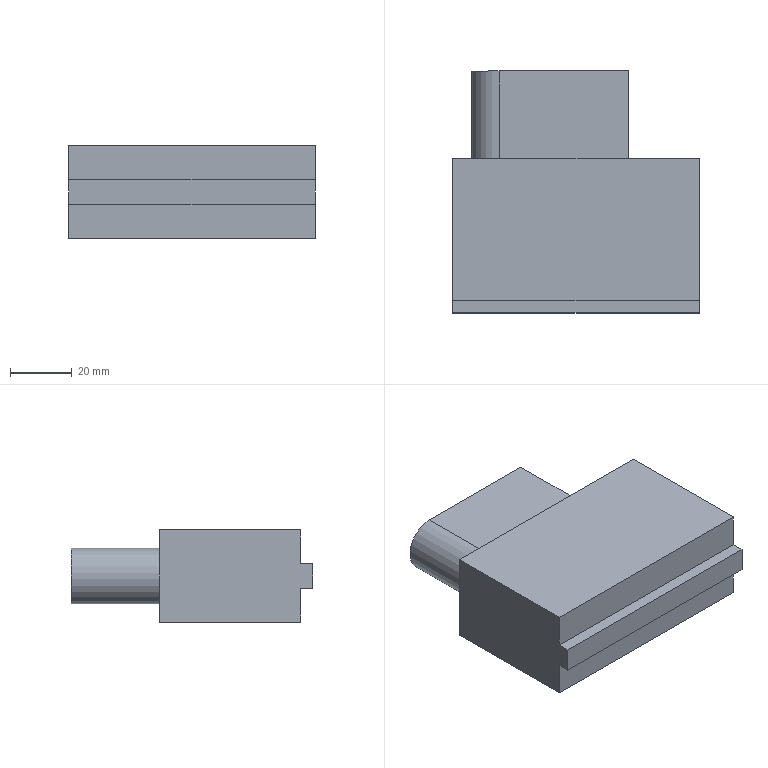Component | SolidWorks | 12ATransverseStraighteningPlatePart-2_12AStraighteningOuterWheel-2_12AOuterSideWheelSeat-1 | 1 solid | 29 faces | box 80 x 78.6 x 30 mm | volume 131776 mm3 | plane 17 | cylinder 8 | cone 4 | commonest cylinder face diameters 8.5 x4 12.5 x3 18 x1 | material Cr12MoV
build123d program:
from build123d import *

# Parameters (mm, degrees)
SKETCH1_W              = 80
SKETCH1_H              = 46
BOSS_EXTRUDE1_DEPTH    = 30
SKETCH2_W              = 80
SKETCH2_H              = 8
BOSS_EXTRUDE2_DEPTH    = 4
BOSS_EXTRUDE3_DEPTH    = 28.6
M10_TAPPED_HOLE1_D     = 8.5
M10_TAPPED_HOLE1_DEPTH = 25
M10_TAPPED_HOLE1_TIP   = 2.554
CUT_EXTRUDE1_DEPTH     = 24


with BuildPart() as part:
    # Sketch1 → Boss-Extrude1 (new body)
    with BuildSketch(Plane.XY):
        with Locations((40, -23)):
            Rectangle(SKETCH1_W, SKETCH1_H)
    extrude(amount=BOSS_EXTRUDE1_DEPTH)

    # Sketch2 → Boss-Extrude2 (add)
    with BuildSketch(Plane(origin=(0, 0, 0), x_dir=(1, 0, 0), z_dir=(0, 1, 0))):
        with Locations((40, -15)):
            Rectangle(SKETCH2_W, SKETCH2_H)
    extrude(amount=BOSS_EXTRUDE2_DEPTH)

    # Sketch3 → Boss-Extrude3 (add)
    with BuildSketch(Plane.XZ.offset(46)):
        with BuildLine():
            Line((57, 24), (57, 6))
            Line((57, 6), (15, 6))
            ThreePointArc((15, 6), (6, 15), (15, 24))
            Line((15, 24), (57, 24))
        make_face()
    extrude(amount=BOSS_EXTRUDE3_DEPTH)

    # M10 Tapped Hole1
    with Locations(Plane(origin=(0, -74.6, 0), x_dir=(-1, 0, 0), z_dir=(0, -1, 0))):
        with Locations((-35, -15), (-15, -15)):
            Hole(M10_TAPPED_HOLE1_D / 2, depth=M10_TAPPED_HOLE1_DEPTH)
            with Locations((0, 0, -(M10_TAPPED_HOLE1_DEPTH + M10_TAPPED_HOLE1_TIP / 2))):  # 118° drill point
                Cone(0, M10_TAPPED_HOLE1_D / 2, M10_TAPPED_HOLE1_TIP, mode=Mode.SUBTRACT)

    # Sketch6 → Cut-Extrude1 (cut)
    with BuildSketch(Plane.XZ.offset(74.6)):
        with BuildLine():
            Line((57, 19.25), (53.083, 19.25))
            ThreePointArc((53.083, 19.25), (42.25, 15), (53.083, 10.75))
            Line((53.083, 10.75), (57, 10.75))
            Line((57, 10.75), (57, 19.25))
        make_face()
    extrude(amount=-CUT_EXTRUDE1_DEPTH, mode=Mode.SUBTRACT)


solid = part.part

# Placed as in the assembly
solid = solid.moved(Location((184.706, 81.46, -62), (180, 0, 0)))
STEP:
#1=CARTESIAN_POINT('',(9.181,5.199,-3.278));
#2=VERTEX_POINT('',#1);
#3=CARTESIAN_POINT('',(9.181,5.199,-2.785));
#4=VERTEX_POINT('',#3);
#5=CARTESIAN_POINT('',(9.181,5.199,-3.031));
#6=DIRECTION('',(-0.,1.,0.));
#7=DIRECTION('',(0.,0.,1.));
#8=AXIS2_PLACEMENT_3D('',#5,#6,#7);
#9=CIRCLE('',#8,0.2461);
#10=EDGE_CURVE('',#2,#4,#9,.T.);
#11=ORIENTED_EDGE('',*,*,#10,.F.);
#12=CARTESIAN_POINT('',(9.181,6.144,-3.278));
#13=VERTEX_POINT('',#12);
#14=CARTESIAN_POINT('',(9.181,5.199,-3.278));
#15=DIRECTION('',(-0.,1.,0.));
#16=VECTOR('',#15,39.37);
#17=LINE('',#14,#16);
#18=EDGE_CURVE('',#2,#13,#17,.T.);
#19=ORIENTED_EDGE('',*,*,#18,.T.);
#20=CARTESIAN_POINT('',(9.181,6.144,-2.785));
#21=VERTEX_POINT('',#20);
#22=CARTESIAN_POINT('',(9.181,6.144,-3.031));
#23=DIRECTION('',(-0.,1.,0.));
#24=DIRECTION('',(0.,0.,1.));
#25=AXIS2_PLACEMENT_3D('',#22,#23,#24);
#26=CIRCLE('',#25,0.2461);
#27=EDGE_CURVE('',#13,#21,#26,.T.);
#28=ORIENTED_EDGE('',*,*,#27,.T.);
#29=CARTESIAN_POINT('',(9.181,5.199,-2.785));
#30=DIRECTION('',(-0.,1.,0.));
#31=VECTOR('',#30,39.37);
#32=LINE('',#29,#31);
#33=EDGE_CURVE('',#4,#21,#32,.T.);
#34=ORIENTED_EDGE('',*,*,#33,.F.);
#35=EDGE_LOOP('',(#11,#19,#28,#34));
#36=FACE_OUTER_BOUND('',#35,.T.);
#37=CARTESIAN_POINT('',(9.181,5.199,-3.031));
#38=DIRECTION('',(-0.,1.,0.));
#39=DIRECTION('',(0.,0.,1.));
#40=AXIS2_PLACEMENT_3D('',#37,#38,#39);
#41=CYLINDRICAL_SURFACE('',#40,0.2461);
#42=ADVANCED_FACE('',(#36),#41,.F.);
#43=CARTESIAN_POINT('',(9.362,5.199,-2.864));
#44=VERTEX_POINT('',#43);
#45=CARTESIAN_POINT('',(9.181,5.199,-3.031));
#46=DIRECTION('',(-0.,1.,0.));
#47=DIRECTION('',(0.,0.,1.));
#48=AXIS2_PLACEMENT_3D('',#45,#46,#47);
#49=CIRCLE('',#48,0.2461);
#50=EDGE_CURVE('',#4,#44,#49,.T.);
#51=ORIENTED_EDGE('',*,*,#50,.F.);
#52=ORIENTED_EDGE('',*,*,#33,.T.);
#53=CARTESIAN_POINT('',(9.362,6.144,-2.864));
#54=VERTEX_POINT('',#53);
#55=CARTESIAN_POINT('',(9.181,6.144,-3.031));
#56=DIRECTION('',(-0.,1.,0.));
#57=DIRECTION('',(0.,0.,1.));
#58=AXIS2_PLACEMENT_3D('',#55,#56,#57);
#59=CIRCLE('',#58,0.2461);
#60=EDGE_CURVE('',#21,#54,#59,.T.);
#61=ORIENTED_EDGE('',*,*,#60,.T.);
#62=CARTESIAN_POINT('',(9.362,5.199,-2.864));
#63=DIRECTION('',(-0.,1.,0.));
#64=VECTOR('',#63,39.37);
#65=LINE('',#62,#64);
#66=EDGE_CURVE('',#44,#54,#65,.T.);
#67=ORIENTED_EDGE('',*,*,#66,.F.);
#68=EDGE_LOOP('',(#51,#52,#61,#67));
#69=FACE_OUTER_BOUND('',#68,.T.);
#70=CARTESIAN_POINT('',(9.181,5.199,-3.031));
#71=DIRECTION('',(-0.,1.,0.));
#72=DIRECTION('',(0.,0.,1.));
#73=AXIS2_PLACEMENT_3D('',#70,#71,#72);
#74=CYLINDRICAL_SURFACE('',#73,0.2461);
#75=ADVANCED_FACE('',(#69),#74,.F.);
#76=CARTESIAN_POINT('',(7.862,5.16,-3.199));
#77=VERTEX_POINT('',#76);
#78=CARTESIAN_POINT('',(7.862,5.16,-2.864));
#79=VERTEX_POINT('',#78);
#80=CARTESIAN_POINT('',(7.862,5.16,-3.031));
#81=DIRECTION('',(-0.,1.,0.));
#82=DIRECTION('',(0.,0.,1.));
#83=AXIS2_PLACEMENT_3D('',#80,#81,#82);
#84=CIRCLE('',#83,0.1673);
#85=EDGE_CURVE('',#77,#79,#84,.T.);
#86=ORIENTED_EDGE('',*,*,#85,.F.);
#87=CARTESIAN_POINT('',(7.862,6.144,-3.199));
#88=VERTEX_POINT('',#87);
#89=CARTESIAN_POINT('',(7.862,6.144,-3.199));
#90=DIRECTION('',(-0.,1.,0.));
#91=VECTOR('',#90,39.37);
#92=LINE('',#89,#91);
#93=EDGE_CURVE('',#77,#88,#92,.T.);
#94=ORIENTED_EDGE('',*,*,#93,.T.);
#95=CARTESIAN_POINT('',(7.862,6.144,-2.864));
#96=VERTEX_POINT('',#95);
#97=CARTESIAN_POINT('',(7.862,6.144,-3.031));
#98=DIRECTION('',(-0.,1.,0.));
#99=DIRECTION('',(0.,0.,1.));
#100=AXIS2_PLACEMENT_3D('',#97,#98,#99);
#101=CIRCLE('',#100,0.1673);
#102=EDGE_CURVE('',#88,#96,#101,.T.);
#103=ORIENTED_EDGE('',*,*,#102,.T.);
#104=CARTESIAN_POINT('',(7.862,6.144,-2.864));
#105=DIRECTION('',(-0.,1.,0.));
#106=VECTOR('',#105,39.37);
#107=LINE('',#104,#106);
#108=EDGE_CURVE('',#79,#96,#107,.T.);
#109=ORIENTED_EDGE('',*,*,#108,.F.);
#110=EDGE_LOOP('',(#86,#94,#103,#109));
#111=FACE_OUTER_BOUND('',#110,.T.);
#112=CARTESIAN_POINT('',(7.862,6.144,-3.031));
#113=DIRECTION('',(-0.,1.,0.));
#114=DIRECTION('',(0.,0.,1.));
#115=AXIS2_PLACEMENT_3D('',#112,#113,#114);
#116=CYLINDRICAL_SURFACE('',#115,0.1673);
#117=ADVANCED_FACE('',(#111),#116,.F.);
#118=CARTESIAN_POINT('',(7.862,5.059,-3.031));
#119=VERTEX_POINT('',#118);
#120=CARTESIAN_POINT('',(7.862,5.16,-2.864));
#121=DIRECTION('',(-0.,0.515,0.8572));
#122=VECTOR('',#121,39.37);
#123=LINE('',#120,#122);
#124=EDGE_CURVE('',#119,#79,#123,.T.);
#125=ORIENTED_EDGE('',*,*,#124,.F.);
#126=CARTESIAN_POINT('',(7.862,5.16,-3.199));
#127=DIRECTION('',(-0.,0.515,-0.8572));
#128=VECTOR('',#127,39.37);
#129=LINE('',#126,#128);
#130=EDGE_CURVE('',#119,#77,#129,.T.);
#131=ORIENTED_EDGE('',*,*,#130,.T.);
#132=ORIENTED_EDGE('',*,*,#85,.T.);
#133=EDGE_LOOP('',(#125,#131,#132));
#134=FACE_OUTER_BOUND('',#133,.T.);
#135=CARTESIAN_POINT('',(7.862,5.16,-3.031));
#136=DIRECTION('',(-0.,1.,0.));
#137=DIRECTION('',(0.,0.,1.));
#138=AXIS2_PLACEMENT_3D('',#135,#136,#137);
#139=CONICAL_SURFACE('',#138,0.1673,1.03);
#140=ADVANCED_FACE('',(#134),#139,.F.);
#141=CARTESIAN_POINT('',(8.65,5.16,-3.199));
#142=VERTEX_POINT('',#141);
#143=CARTESIAN_POINT('',(8.65,5.16,-2.864));
#144=VERTEX_POINT('',#143);
#145=CARTESIAN_POINT('',(8.65,5.16,-3.031));
#146=DIRECTION('',(-0.,1.,0.));
#147=DIRECTION('',(0.,0.,1.));
#148=AXIS2_PLACEMENT_3D('',#145,#146,#147);
#149=CIRCLE('',#148,0.1673);
#150=EDGE_CURVE('',#142,#144,#149,.T.);
#151=ORIENTED_EDGE('',*,*,#150,.F.);
#152=CARTESIAN_POINT('',(8.65,6.144,-3.199));
#153=VERTEX_POINT('',#152);
#154=CARTESIAN_POINT('',(8.65,6.144,-3.199));
#155=DIRECTION('',(-0.,1.,0.));
#156=VECTOR('',#155,39.37);
#157=LINE('',#154,#156);
#158=EDGE_CURVE('',#142,#153,#157,.T.);
#159=ORIENTED_EDGE('',*,*,#158,.T.);
#160=CARTESIAN_POINT('',(8.65,6.144,-2.864));
#161=VERTEX_POINT('',#160);
#162=CARTESIAN_POINT('',(8.65,6.144,-3.031));
#163=DIRECTION('',(-0.,1.,0.));
#164=DIRECTION('',(0.,0.,1.));
#165=AXIS2_PLACEMENT_3D('',#162,#163,#164);
#166=CIRCLE('',#165,0.1673);
#167=EDGE_CURVE('',#153,#161,#166,.T.);
#168=ORIENTED_EDGE('',*,*,#167,.T.);
#169=CARTESIAN_POINT('',(8.65,6.144,-2.864));
#170=DIRECTION('',(-0.,1.,0.));
#171=VECTOR('',#170,39.37);
#172=LINE('',#169,#171);
#173=EDGE_CURVE('',#144,#161,#172,.T.);
#174=ORIENTED_EDGE('',*,*,#173,.F.);
#175=EDGE_LOOP('',(#151,#159,#168,#174));
#176=FACE_OUTER_BOUND('',#175,.T.);
#177=CARTESIAN_POINT('',(8.65,6.144,-3.031));
#178=DIRECTION('',(-0.,1.,0.));
#179=DIRECTION('',(0.,0.,1.));
#180=AXIS2_PLACEMENT_3D('',#177,#178,#179);
#181=CYLINDRICAL_SURFACE('',#180,0.1673);
#182=ADVANCED_FACE('',(#176),#181,.F.);
#183=CARTESIAN_POINT('',(8.65,5.059,-3.031));
#184=VERTEX_POINT('',#183);
#185=CARTESIAN_POINT('',(8.65,5.16,-2.864));
#186=DIRECTION('',(-0.,0.515,0.8572));
#187=VECTOR('',#186,39.37);
#188=LINE('',#185,#187);
#189=EDGE_CURVE('',#184,#144,#188,.T.);
#190=ORIENTED_EDGE('',*,*,#189,.F.);
#191=CARTESIAN_POINT('',(8.65,5.16,-3.199));
#192=DIRECTION('',(-0.,0.515,-0.8572));
#193=VECTOR('',#192,39.37);
#194=LINE('',#191,#193);
#195=EDGE_CURVE('',#184,#142,#194,.T.);
#196=ORIENTED_EDGE('',*,*,#195,.T.);
#197=ORIENTED_EDGE('',*,*,#150,.T.);
#198=EDGE_LOOP('',(#190,#196,#197));
#199=FACE_OUTER_BOUND('',#198,.T.);
#200=CARTESIAN_POINT('',(8.65,5.16,-3.031));
#201=DIRECTION('',(-0.,1.,0.));
#202=DIRECTION('',(0.,0.,1.));
#203=AXIS2_PLACEMENT_3D('',#200,#201,#202);
#204=CONICAL_SURFACE('',#203,0.1673,1.03);
#205=ADVANCED_FACE('',(#199),#204,.F.);
#206=CARTESIAN_POINT('',(7.272,5.018,-2.441));
#207=VERTEX_POINT('',#206);
#208=CARTESIAN_POINT('',(10.422,5.018,-2.441));
#209=VERTEX_POINT('',#208);
#210=CARTESIAN_POINT('',(7.272,5.018,-2.441));
#211=DIRECTION('',(1.,0.,-0.));
#212=VECTOR('',#211,39.37);
#213=LINE('',#210,#212);
#214=EDGE_CURVE('',#207,#209,#213,.T.);
#215=ORIENTED_EDGE('',*,*,#214,.T.);
#216=CARTESIAN_POINT('',(10.422,5.018,-3.622));
#217=VERTEX_POINT('',#216);
#218=CARTESIAN_POINT('',(10.422,5.018,-3.622));
#219=DIRECTION('',(0.,0.,1.));
#220=VECTOR('',#219,39.37);
#221=LINE('',#218,#220);
#222=EDGE_CURVE('',#217,#209,#221,.T.);
#223=ORIENTED_EDGE('',*,*,#222,.F.);
#224=CARTESIAN_POINT('',(7.272,5.018,-3.622));
#225=VERTEX_POINT('',#224);
#226=CARTESIAN_POINT('',(7.272,5.018,-3.622));
#227=DIRECTION('',(1.,0.,-0.));
#228=VECTOR('',#227,39.37);
#229=LINE('',#226,#228);
#230=EDGE_CURVE('',#225,#217,#229,.T.);
#231=ORIENTED_EDGE('',*,*,#230,.F.);
#232=CARTESIAN_POINT('',(7.272,5.018,-3.622));
#233=DIRECTION('',(0.,0.,1.));
#234=VECTOR('',#233,39.37);
#235=LINE('',#232,#234);
#236=EDGE_CURVE('',#225,#207,#235,.T.);
#237=ORIENTED_EDGE('',*,*,#236,.T.);
#238=EDGE_LOOP('',(#215,#223,#231,#237));
#239=FACE_OUTER_BOUND('',#238,.T.);
#240=CARTESIAN_POINT('',(7.862,5.018,-3.386));
#241=VERTEX_POINT('',#240);
#242=CARTESIAN_POINT('',(7.862,5.018,-2.677));
#243=VERTEX_POINT('',#242);
#244=CARTESIAN_POINT('',(7.862,5.018,-3.031));
#245=DIRECTION('',(-0.,1.,0.));
#246=DIRECTION('',(0.,0.,1.));
#247=AXIS2_PLACEMENT_3D('',#244,#245,#246);
#248=CIRCLE('',#247,0.3543);
#249=EDGE_CURVE('',#241,#243,#248,.T.);
#250=ORIENTED_EDGE('',*,*,#249,.F.);
#251=CARTESIAN_POINT('',(9.516,5.018,-3.386));
#252=VERTEX_POINT('',#251);
#253=CARTESIAN_POINT('',(7.862,5.018,-3.386));
#254=DIRECTION('',(-1.,-0.,0.));
#255=VECTOR('',#254,39.37);
#256=LINE('',#253,#255);
#257=EDGE_CURVE('',#252,#241,#256,.T.);
#258=ORIENTED_EDGE('',*,*,#257,.F.);
#259=CARTESIAN_POINT('',(9.516,5.018,-2.677));
#260=VERTEX_POINT('',#259);
#261=CARTESIAN_POINT('',(9.516,5.018,-3.386));
#262=DIRECTION('',(0.,0.,-1.));
#263=VECTOR('',#262,39.37);
#264=LINE('',#261,#263);
#265=EDGE_CURVE('',#260,#252,#264,.T.);
#266=ORIENTED_EDGE('',*,*,#265,.F.);
#267=CARTESIAN_POINT('',(7.862,5.018,-2.677));
#268=DIRECTION('',(1.,0.,-0.));
#269=VECTOR('',#268,39.37);
#270=LINE('',#267,#269);
#271=EDGE_CURVE('',#243,#260,#270,.T.);
#272=ORIENTED_EDGE('',*,*,#271,.F.);
#273=EDGE_LOOP('',(#250,#258,#266,#272));
#274=FACE_BOUND('',#273,.T.);
#275=CARTESIAN_POINT('',(7.272,5.018,-3.622));
#276=DIRECTION('',(0.,-1.,-0.));
#277=DIRECTION('',(-0.,-0.,-1.));
#278=AXIS2_PLACEMENT_3D('',#275,#276,#277);
#279=PLANE('',#278);
#280=ADVANCED_FACE('',(#239,#274),#279,.F.);
#281=CARTESIAN_POINT('',(10.422,3.207,-2.874));
#282=VERTEX_POINT('',#281);
#283=CARTESIAN_POINT('',(7.272,3.207,-2.874));
#284=VERTEX_POINT('',#283);
#285=CARTESIAN_POINT('',(7.272,3.207,-2.874));
#286=DIRECTION('',(-1.,-0.,0.));
#287=VECTOR('',#286,39.37);
#288=LINE('',#285,#287);
#289=EDGE_CURVE('',#282,#284,#288,.T.);
#290=ORIENTED_EDGE('',*,*,#289,.F.);
#291=CARTESIAN_POINT('',(10.422,3.207,-2.441));
#292=VERTEX_POINT('',#291);
#293=CARTESIAN_POINT('',(10.422,3.207,-3.622));
#294=DIRECTION('',(0.,0.,1.));
#295=VECTOR('',#294,39.37);
#296=LINE('',#293,#295);
#297=EDGE_CURVE('',#282,#292,#296,.T.);
#298=ORIENTED_EDGE('',*,*,#297,.T.);
#299=CARTESIAN_POINT('',(7.272,3.207,-2.441));
#300=VERTEX_POINT('',#299);
#301=CARTESIAN_POINT('',(7.272,3.207,-2.441));
#302=DIRECTION('',(-1.,-0.,0.));
#303=VECTOR('',#302,39.37);
#304=LINE('',#301,#303);
#305=EDGE_CURVE('',#292,#300,#304,.T.);
#306=ORIENTED_EDGE('',*,*,#305,.T.);
#307=CARTESIAN_POINT('',(7.272,3.207,-3.622));
#308=DIRECTION('',(0.,0.,1.));
#309=VECTOR('',#308,39.37);
#310=LINE('',#307,#309);
#311=EDGE_CURVE('',#284,#300,#310,.T.);
#312=ORIENTED_EDGE('',*,*,#311,.F.);
#313=EDGE_LOOP('',(#290,#298,#306,#312));
#314=FACE_OUTER_BOUND('',#313,.T.);
#315=CARTESIAN_POINT('',(7.272,3.207,-3.622));
#316=DIRECTION('',(-0.,1.,0.));
#317=DIRECTION('',(0.,0.,1.));
#318=AXIS2_PLACEMENT_3D('',#315,#316,#317);
#319=PLANE('',#318);
#320=ADVANCED_FACE('',(#314),#319,.F.);
#321=CARTESIAN_POINT('',(7.272,3.207,-3.189));
#322=VERTEX_POINT('',#321);
#323=CARTESIAN_POINT('',(10.422,3.207,-3.189));
#324=VERTEX_POINT('',#323);
#325=CARTESIAN_POINT('',(7.272,3.207,-3.189));
#326=DIRECTION('',(1.,0.,-0.));
#327=VECTOR('',#326,39.37);
#328=LINE('',#325,#327);
#329=EDGE_CURVE('',#322,#324,#328,.T.);
#330=ORIENTED_EDGE('',*,*,#329,.F.);
#331=CARTESIAN_POINT('',(7.272,3.207,-3.622));
#332=VERTEX_POINT('',#331);
#333=CARTESIAN_POINT('',(7.272,3.207,-3.622));
#334=DIRECTION('',(0.,0.,1.));
#335=VECTOR('',#334,39.37);
#336=LINE('',#333,#335);
#337=EDGE_CURVE('',#332,#322,#336,.T.);
#338=ORIENTED_EDGE('',*,*,#337,.F.);
#339=CARTESIAN_POINT('',(10.422,3.207,-3.622));
#340=VERTEX_POINT('',#339);
#341=CARTESIAN_POINT('',(7.272,3.207,-3.622));
#342=DIRECTION('',(-1.,-0.,0.));
#343=VECTOR('',#342,39.37);
#344=LINE('',#341,#343);
#345=EDGE_CURVE('',#340,#332,#344,.T.);
#346=ORIENTED_EDGE('',*,*,#345,.F.);
#347=CARTESIAN_POINT('',(10.422,3.207,-3.622));
#348=DIRECTION('',(0.,0.,1.));
#349=VECTOR('',#348,39.37);
#350=LINE('',#347,#349);
#351=EDGE_CURVE('',#340,#324,#350,.T.);
#352=ORIENTED_EDGE('',*,*,#351,.T.);
#353=EDGE_LOOP('',(#330,#338,#346,#352));
#354=FACE_OUTER_BOUND('',#353,.T.);
#355=CARTESIAN_POINT('',(7.272,3.207,-3.622));
#356=DIRECTION('',(-0.,1.,0.));
#357=DIRECTION('',(0.,0.,1.));
#358=AXIS2_PLACEMENT_3D('',#355,#356,#357);
#359=PLANE('',#358);
#360=ADVANCED_FACE('',(#354),#359,.F.);
#361=CARTESIAN_POINT('',(7.272,3.207,-2.441));
#362=DIRECTION('',(-0.,1.,-0.));
#363=VECTOR('',#362,39.37);
#364=LINE('',#361,#363);
#365=EDGE_CURVE('',#300,#207,#364,.T.);
#366=ORIENTED_EDGE('',*,*,#365,.T.);
#367=ORIENTED_EDGE('',*,*,#236,.F.);
#368=CARTESIAN_POINT('',(7.272,3.207,-3.622));
#369=DIRECTION('',(-0.,1.,-0.));
#370=VECTOR('',#369,39.37);
#371=LINE('',#368,#370);
#372=EDGE_CURVE('',#332,#225,#371,.T.);
#373=ORIENTED_EDGE('',*,*,#372,.F.);
#374=ORIENTED_EDGE('',*,*,#337,.T.);
#375=CARTESIAN_POINT('',(7.272,3.05,-3.189));
#376=VERTEX_POINT('',#375);
#377=CARTESIAN_POINT('',(7.272,3.05,-3.189));
#378=DIRECTION('',(-0.,1.,0.));
#379=VECTOR('',#378,39.37);
#380=LINE('',#377,#379);
#381=EDGE_CURVE('',#376,#322,#380,.T.);
#382=ORIENTED_EDGE('',*,*,#381,.F.);
#383=CARTESIAN_POINT('',(7.272,3.05,-2.874));
#384=VERTEX_POINT('',#383);
#385=CARTESIAN_POINT('',(7.272,3.05,-2.874));
#386=DIRECTION('',(0.,0.,-1.));
#387=VECTOR('',#386,39.37);
#388=LINE('',#385,#387);
#389=EDGE_CURVE('',#384,#376,#388,.T.);
#390=ORIENTED_EDGE('',*,*,#389,.F.);
#391=CARTESIAN_POINT('',(7.272,3.05,-2.874));
#392=DIRECTION('',(-0.,1.,0.));
#393=VECTOR('',#392,39.37);
#394=LINE('',#391,#393);
#395=EDGE_CURVE('',#384,#284,#394,.T.);
#396=ORIENTED_EDGE('',*,*,#395,.T.);
#397=ORIENTED_EDGE('',*,*,#311,.T.);
#398=EDGE_LOOP('',(#366,#367,#373,#374,#382,#390,#396,#397));
#399=FACE_OUTER_BOUND('',#398,.T.);
#400=CARTESIAN_POINT('',(7.272,3.207,-3.622));
#401=DIRECTION('',(1.,0.,-0.));
#402=DIRECTION('',(0.,-1.,0.));
#403=AXIS2_PLACEMENT_3D('',#400,#401,#402);
#404=PLANE('',#403);
#405=ADVANCED_FACE('',(#399),#404,.F.);
#406=CARTESIAN_POINT('',(10.422,3.207,-2.441));
#407=DIRECTION('',(0.,-1.,0.));
#408=VECTOR('',#407,39.37);
#409=LINE('',#406,#408);
#410=EDGE_CURVE('',#209,#292,#409,.T.);
#411=ORIENTED_EDGE('',*,*,#410,.T.);
#412=ORIENTED_EDGE('',*,*,#297,.F.);
#413=CARTESIAN_POINT('',(10.422,3.05,-2.874));
#414=VERTEX_POINT('',#413);
#415=CARTESIAN_POINT('',(10.422,3.05,-2.874));
#416=DIRECTION('',(-0.,1.,0.));
#417=VECTOR('',#416,39.37);
#418=LINE('',#415,#417);
#419=EDGE_CURVE('',#414,#282,#418,.T.);
#420=ORIENTED_EDGE('',*,*,#419,.F.);
#421=CARTESIAN_POINT('',(10.422,3.05,-3.189));
#422=VERTEX_POINT('',#421);
#423=CARTESIAN_POINT('',(10.422,3.05,-2.874));
#424=DIRECTION('',(0.,0.,1.));
#425=VECTOR('',#424,39.37);
#426=LINE('',#423,#425);
#427=EDGE_CURVE('',#422,#414,#426,.T.);
#428=ORIENTED_EDGE('',*,*,#427,.F.);
#429=CARTESIAN_POINT('',(10.422,3.05,-3.189));
#430=DIRECTION('',(-0.,1.,0.));
#431=VECTOR('',#430,39.37);
#432=LINE('',#429,#431);
#433=EDGE_CURVE('',#422,#324,#432,.T.);
#434=ORIENTED_EDGE('',*,*,#433,.T.);
#435=ORIENTED_EDGE('',*,*,#351,.F.);
#436=CARTESIAN_POINT('',(10.422,3.207,-3.622));
#437=DIRECTION('',(0.,-1.,0.));
#438=VECTOR('',#437,39.37);
#439=LINE('',#436,#438);
#440=EDGE_CURVE('',#217,#340,#439,.T.);
#441=ORIENTED_EDGE('',*,*,#440,.F.);
#442=ORIENTED_EDGE('',*,*,#222,.T.);
#443=EDGE_LOOP('',(#411,#412,#420,#428,#434,#435,#441,#442));
#444=FACE_OUTER_BOUND('',#443,.T.);
#445=CARTESIAN_POINT('',(10.422,3.207,-3.622));
#446=DIRECTION('',(-1.,-0.,0.));
#447=DIRECTION('',(-0.,1.,-0.));
#448=AXIS2_PLACEMENT_3D('',#445,#446,#447);
#449=PLANE('',#448);
#450=ADVANCED_FACE('',(#444),#449,.F.);
#451=ORIENTED_EDGE('',*,*,#372,.T.);
#452=ORIENTED_EDGE('',*,*,#230,.T.);
#453=ORIENTED_EDGE('',*,*,#440,.T.);
#454=ORIENTED_EDGE('',*,*,#345,.T.);
#455=EDGE_LOOP('',(#451,#452,#453,#454));
#456=FACE_OUTER_BOUND('',#455,.T.);
#457=CARTESIAN_POINT('',(7.272,3.207,-3.622));
#458=DIRECTION('',(-0.,-0.,-1.));
#459=DIRECTION('',(1.,0.,-0.));
#460=AXIS2_PLACEMENT_3D('',#457,#458,#459);
#461=PLANE('',#460);
#462=ADVANCED_FACE('',(#456),#461,.T.);
#463=ORIENTED_EDGE('',*,*,#365,.F.);
#464=ORIENTED_EDGE('',*,*,#305,.F.);
#465=ORIENTED_EDGE('',*,*,#410,.F.);
#466=ORIENTED_EDGE('',*,*,#214,.F.);
#467=EDGE_LOOP('',(#463,#464,#465,#466));
#468=FACE_OUTER_BOUND('',#467,.T.);
#469=CARTESIAN_POINT('',(7.272,3.207,-2.441));
#470=DIRECTION('',(-0.,-0.,-1.));
#471=DIRECTION('',(1.,0.,-0.));
#472=AXIS2_PLACEMENT_3D('',#469,#470,#471);
#473=PLANE('',#472);
#474=ADVANCED_FACE('',(#468),#473,.F.);
#475=ORIENTED_EDGE('',*,*,#329,.T.);
#476=ORIENTED_EDGE('',*,*,#433,.F.);
#477=CARTESIAN_POINT('',(7.272,3.05,-3.189));
#478=DIRECTION('',(1.,0.,-0.));
#479=VECTOR('',#478,39.37);
#480=LINE('',#477,#479);
#481=EDGE_CURVE('',#376,#422,#480,.T.);
#482=ORIENTED_EDGE('',*,*,#481,.F.);
#483=ORIENTED_EDGE('',*,*,#381,.T.);
#484=EDGE_LOOP('',(#475,#476,#482,#483));
#485=FACE_OUTER_BOUND('',#484,.T.);
#486=CARTESIAN_POINT('',(7.272,3.05,-3.189));
#487=DIRECTION('',(0.,0.,1.));
#488=DIRECTION('',(-1.,-0.,0.));
#489=AXIS2_PLACEMENT_3D('',#486,#487,#488);
#490=PLANE('',#489);
#491=ADVANCED_FACE('',(#485),#490,.F.);
#492=ORIENTED_EDGE('',*,*,#289,.T.);
#493=ORIENTED_EDGE('',*,*,#395,.F.);
#494=CARTESIAN_POINT('',(7.272,3.05,-2.874));
#495=DIRECTION('',(-1.,-0.,0.));
#496=VECTOR('',#495,39.37);
#497=LINE('',#494,#496);
#498=EDGE_CURVE('',#414,#384,#497,.T.);
#499=ORIENTED_EDGE('',*,*,#498,.F.);
#500=ORIENTED_EDGE('',*,*,#419,.T.);
#501=EDGE_LOOP('',(#492,#493,#499,#500));
#502=FACE_OUTER_BOUND('',#501,.T.);
#503=CARTESIAN_POINT('',(7.272,3.05,-2.874));
#504=DIRECTION('',(-0.,-0.,-1.));
#505=DIRECTION('',(1.,0.,-0.));
#506=AXIS2_PLACEMENT_3D('',#503,#504,#505);
#507=PLANE('',#506);
#508=ADVANCED_FACE('',(#502),#507,.F.);
#509=ORIENTED_EDGE('',*,*,#389,.T.);
#510=ORIENTED_EDGE('',*,*,#481,.T.);
#511=ORIENTED_EDGE('',*,*,#427,.T.);
#512=ORIENTED_EDGE('',*,*,#498,.T.);
#513=EDGE_LOOP('',(#509,#510,#511,#512));
#514=FACE_OUTER_BOUND('',#513,.T.);
#515=CARTESIAN_POINT('',(7.272,3.05,-2.441));
#516=DIRECTION('',(0.,-1.,-0.));
#517=DIRECTION('',(-0.,-0.,-1.));
#518=AXIS2_PLACEMENT_3D('',#515,#516,#517);
#519=PLANE('',#518);
#520=ADVANCED_FACE('',(#514),#519,.T.);
#521=ORIENTED_EDGE('',*,*,#249,.T.);
#522=CARTESIAN_POINT('',(7.862,6.144,-2.677));
#523=VERTEX_POINT('',#522);
#524=CARTESIAN_POINT('',(7.862,6.144,-2.677));
#525=DIRECTION('',(0.,-1.,-0.));
#526=VECTOR('',#525,39.37);
#527=LINE('',#524,#526);
#528=EDGE_CURVE('',#523,#243,#527,.T.);
#529=ORIENTED_EDGE('',*,*,#528,.F.);
#530=CARTESIAN_POINT('',(7.862,6.144,-3.386));
#531=VERTEX_POINT('',#530);
#532=CARTESIAN_POINT('',(7.862,6.144,-3.031));
#533=DIRECTION('',(-0.,1.,0.));
#534=DIRECTION('',(0.,0.,1.));
#535=AXIS2_PLACEMENT_3D('',#532,#533,#534);
#536=CIRCLE('',#535,0.3543);
#537=EDGE_CURVE('',#531,#523,#536,.T.);
#538=ORIENTED_EDGE('',*,*,#537,.F.);
#539=CARTESIAN_POINT('',(7.862,6.144,-3.386));
#540=DIRECTION('',(0.,-1.,-0.));
#541=VECTOR('',#540,39.37);
#542=LINE('',#539,#541);
#543=EDGE_CURVE('',#531,#241,#542,.T.);
#544=ORIENTED_EDGE('',*,*,#543,.T.);
#545=EDGE_LOOP('',(#521,#529,#538,#544));
#546=FACE_OUTER_BOUND('',#545,.T.);
#547=CARTESIAN_POINT('',(7.862,6.144,-3.031));
#548=DIRECTION('',(0.,-1.,-0.));
#549=DIRECTION('',(0.,0.,-1.));
#550=AXIS2_PLACEMENT_3D('',#547,#548,#549);
#551=CYLINDRICAL_SURFACE('',#550,0.3543);
#552=ADVANCED_FACE('',(#546),#551,.T.);
#553=ORIENTED_EDGE('',*,*,#271,.T.);
#554=CARTESIAN_POINT('',(9.516,6.144,-2.677));
#555=VERTEX_POINT('',#554);
#556=CARTESIAN_POINT('',(9.516,6.144,-2.677));
#557=DIRECTION('',(0.,-1.,-0.));
#558=VECTOR('',#557,39.37);
#559=LINE('',#556,#558);
#560=EDGE_CURVE('',#555,#260,#559,.T.);
#561=ORIENTED_EDGE('',*,*,#560,.F.);
#562=CARTESIAN_POINT('',(7.862,6.144,-2.677));
#563=DIRECTION('',(1.,0.,-0.));
#564=VECTOR('',#563,39.37);
#565=LINE('',#562,#564);
#566=EDGE_CURVE('',#523,#555,#565,.T.);
#567=ORIENTED_EDGE('',*,*,#566,.F.);
#568=ORIENTED_EDGE('',*,*,#528,.T.);
#569=EDGE_LOOP('',(#553,#561,#567,#568));
#570=FACE_OUTER_BOUND('',#569,.T.);
#571=CARTESIAN_POINT('',(7.862,6.144,-2.677));
#572=DIRECTION('',(-0.,-0.,-1.));
#573=DIRECTION('',(1.,0.,-0.));
#574=AXIS2_PLACEMENT_3D('',#571,#572,#573);
#575=PLANE('',#574);
#576=ADVANCED_FACE('',(#570),#575,.F.);
#577=CARTESIAN_POINT('',(9.516,5.199,-2.864));
#578=VERTEX_POINT('',#577);
#579=CARTESIAN_POINT('',(9.516,5.199,-3.199));
#580=VERTEX_POINT('',#579);
#581=CARTESIAN_POINT('',(9.516,5.199,-3.199));
#582=DIRECTION('',(-0.,-0.,-1.));
#583=VECTOR('',#582,39.37);
#584=LINE('',#581,#583);
#585=EDGE_CURVE('',#578,#580,#584,.T.);
#586=ORIENTED_EDGE('',*,*,#585,.F.);
#587=CARTESIAN_POINT('',(9.516,6.144,-2.864));
#588=VERTEX_POINT('',#587);
#589=CARTESIAN_POINT('',(9.516,5.199,-2.864));
#590=DIRECTION('',(-0.,1.,0.));
#591=VECTOR('',#590,39.37);
#592=LINE('',#589,#591);
#593=EDGE_CURVE('',#578,#588,#592,.T.);
#594=ORIENTED_EDGE('',*,*,#593,.T.);
#595=CARTESIAN_POINT('',(9.516,6.144,-3.386));
#596=DIRECTION('',(0.,0.,-1.));
#597=VECTOR('',#596,39.37);
#598=LINE('',#595,#597);
#599=EDGE_CURVE('',#555,#588,#598,.T.);
#600=ORIENTED_EDGE('',*,*,#599,.F.);
#601=ORIENTED_EDGE('',*,*,#560,.T.);
#602=ORIENTED_EDGE('',*,*,#265,.T.);
#603=CARTESIAN_POINT('',(9.516,6.144,-3.386));
#604=VERTEX_POINT('',#603);
#605=CARTESIAN_POINT('',(9.516,6.144,-3.386));
#606=DIRECTION('',(0.,-1.,-0.));
#607=VECTOR('',#606,39.37);
#608=LINE('',#605,#607);
#609=EDGE_CURVE('',#604,#252,#608,.T.);
#610=ORIENTED_EDGE('',*,*,#609,.F.);
#611=CARTESIAN_POINT('',(9.516,6.144,-3.199));
#612=VERTEX_POINT('',#611);
#613=CARTESIAN_POINT('',(9.516,6.144,-3.386));
#614=DIRECTION('',(0.,0.,-1.));
#615=VECTOR('',#614,39.37);
#616=LINE('',#613,#615);
#617=EDGE_CURVE('',#612,#604,#616,.T.);
#618=ORIENTED_EDGE('',*,*,#617,.F.);
#619=CARTESIAN_POINT('',(9.516,5.199,-3.199));
#620=DIRECTION('',(-0.,1.,0.));
#621=VECTOR('',#620,39.37);
#622=LINE('',#619,#621);
#623=EDGE_CURVE('',#580,#612,#622,.T.);
#624=ORIENTED_EDGE('',*,*,#623,.F.);
#625=EDGE_LOOP('',(#586,#594,#600,#601,#602,#610,#618,#624));
#626=FACE_OUTER_BOUND('',#625,.T.);
#627=CARTESIAN_POINT('',(9.516,6.144,-3.386));
#628=DIRECTION('',(-1.,-0.,-0.));
#629=DIRECTION('',(0.,0.,-1.));
#630=AXIS2_PLACEMENT_3D('',#627,#628,#629);
#631=PLANE('',#630);
#632=ADVANCED_FACE('',(#626),#631,.F.);
#633=ORIENTED_EDGE('',*,*,#257,.T.);
#634=ORIENTED_EDGE('',*,*,#543,.F.);
#635=CARTESIAN_POINT('',(7.862,6.144,-3.386));
#636=DIRECTION('',(-1.,-0.,0.));
#637=VECTOR('',#636,39.37);
#638=LINE('',#635,#637);
#639=EDGE_CURVE('',#604,#531,#638,.T.);
#640=ORIENTED_EDGE('',*,*,#639,.F.);
#641=ORIENTED_EDGE('',*,*,#609,.T.);
#642=EDGE_LOOP('',(#633,#634,#640,#641));
#643=FACE_OUTER_BOUND('',#642,.T.);
#644=CARTESIAN_POINT('',(7.862,6.144,-3.386));
#645=DIRECTION('',(0.,0.,1.));
#646=DIRECTION('',(-1.,-0.,0.));
#647=AXIS2_PLACEMENT_3D('',#644,#645,#646);
#648=PLANE('',#647);
#649=ADVANCED_FACE('',(#643),#648,.F.);
#650=CARTESIAN_POINT('',(9.516,6.144,-2.864));
#651=DIRECTION('',(1.,0.,-0.));
#652=VECTOR('',#651,39.37);
#653=LINE('',#650,#652);
#654=EDGE_CURVE('',#54,#588,#653,.T.);
#655=ORIENTED_EDGE('',*,*,#654,.F.);
#656=ORIENTED_EDGE('',*,*,#60,.F.);
#657=ORIENTED_EDGE('',*,*,#27,.F.);
#658=CARTESIAN_POINT('',(9.362,6.144,-3.199));
#659=VERTEX_POINT('',#658);
#660=CARTESIAN_POINT('',(9.181,6.144,-3.031));
#661=DIRECTION('',(-0.,1.,0.));
#662=DIRECTION('',(0.,0.,1.));
#663=AXIS2_PLACEMENT_3D('',#660,#661,#662);
#664=CIRCLE('',#663,0.2461);
#665=EDGE_CURVE('',#659,#13,#664,.T.);
#666=ORIENTED_EDGE('',*,*,#665,.F.);
#667=CARTESIAN_POINT('',(9.516,6.144,-3.199));
#668=DIRECTION('',(-1.,-0.,0.));
#669=VECTOR('',#668,39.37);
#670=LINE('',#667,#669);
#671=EDGE_CURVE('',#612,#659,#670,.T.);
#672=ORIENTED_EDGE('',*,*,#671,.F.);
#673=ORIENTED_EDGE('',*,*,#617,.T.);
#674=ORIENTED_EDGE('',*,*,#639,.T.);
#675=ORIENTED_EDGE('',*,*,#537,.T.);
#676=ORIENTED_EDGE('',*,*,#566,.T.);
#677=ORIENTED_EDGE('',*,*,#599,.T.);
#678=EDGE_LOOP('',(#655,#656,#657,#666,#672,#673,#674,#675,#676,#677));
#679=FACE_OUTER_BOUND('',#678,.T.);
#680=CARTESIAN_POINT('',(7.862,6.144,-3.031));
#681=DIRECTION('',(-0.,1.,0.));
#682=DIRECTION('',(0.,0.,1.));
#683=AXIS2_PLACEMENT_3D('',#680,#681,#682);
#684=CIRCLE('',#683,0.1673);
#685=EDGE_CURVE('',#96,#88,#684,.T.);
#686=ORIENTED_EDGE('',*,*,#685,.F.);
#687=ORIENTED_EDGE('',*,*,#102,.F.);
#688=EDGE_LOOP('',(#686,#687));
#689=FACE_BOUND('',#688,.T.);
#690=CARTESIAN_POINT('',(8.65,6.144,-3.031));
#691=DIRECTION('',(-0.,1.,0.));
#692=DIRECTION('',(0.,0.,1.));
#693=AXIS2_PLACEMENT_3D('',#690,#691,#692);
#694=CIRCLE('',#693,0.1673);
#695=EDGE_CURVE('',#161,#153,#694,.T.);
#696=ORIENTED_EDGE('',*,*,#695,.F.);
#697=ORIENTED_EDGE('',*,*,#167,.F.);
#698=EDGE_LOOP('',(#696,#697));
#699=FACE_BOUND('',#698,.T.);
#700=CARTESIAN_POINT('',(7.862,6.144,-3.031));
#701=DIRECTION('',(-0.,1.,0.));
#702=DIRECTION('',(0.,0.,1.));
#703=AXIS2_PLACEMENT_3D('',#700,#701,#702);
#704=PLANE('',#703);
#705=ADVANCED_FACE('',(#679,#689,#699),#704,.T.);
#706=ORIENTED_EDGE('',*,*,#195,.F.);
#707=ORIENTED_EDGE('',*,*,#189,.T.);
#708=CARTESIAN_POINT('',(8.65,5.16,-3.031));
#709=DIRECTION('',(-0.,1.,0.));
#710=DIRECTION('',(0.,0.,1.));
#711=AXIS2_PLACEMENT_3D('',#708,#709,#710);
#712=CIRCLE('',#711,0.1673);
#713=EDGE_CURVE('',#144,#142,#712,.T.);
#714=ORIENTED_EDGE('',*,*,#713,.T.);
#715=EDGE_LOOP('',(#706,#707,#714));
#716=FACE_OUTER_BOUND('',#715,.T.);
#717=CARTESIAN_POINT('',(8.65,5.16,-3.031));
#718=DIRECTION('',(-0.,1.,0.));
#719=DIRECTION('',(0.,0.,1.));
#720=AXIS2_PLACEMENT_3D('',#717,#718,#719);
#721=CONICAL_SURFACE('',#720,0.1673,1.03);
#722=ADVANCED_FACE('',(#716),#721,.F.);
#723=ORIENTED_EDGE('',*,*,#158,.F.);
#724=ORIENTED_EDGE('',*,*,#713,.F.);
#725=ORIENTED_EDGE('',*,*,#173,.T.);
#726=ORIENTED_EDGE('',*,*,#695,.T.);
#727=EDGE_LOOP('',(#723,#724,#725,#726));
#728=FACE_OUTER_BOUND('',#727,.T.);
#729=CARTESIAN_POINT('',(8.65,6.144,-3.031));
#730=DIRECTION('',(-0.,1.,0.));
#731=DIRECTION('',(0.,0.,1.));
#732=AXIS2_PLACEMENT_3D('',#729,#730,#731);
#733=CYLINDRICAL_SURFACE('',#732,0.1673);
#734=ADVANCED_FACE('',(#728),#733,.F.);
#735=ORIENTED_EDGE('',*,*,#130,.F.);
#736=ORIENTED_EDGE('',*,*,#124,.T.);
#737=CARTESIAN_POINT('',(7.862,5.16,-3.031));
#738=DIRECTION('',(-0.,1.,0.));
#739=DIRECTION('',(0.,0.,1.));
#740=AXIS2_PLACEMENT_3D('',#737,#738,#739);
#741=CIRCLE('',#740,0.1673);
#742=EDGE_CURVE('',#79,#77,#741,.T.);
#743=ORIENTED_EDGE('',*,*,#742,.T.);
#744=EDGE_LOOP('',(#735,#736,#743));
#745=FACE_OUTER_BOUND('',#744,.T.);
#746=CARTESIAN_POINT('',(7.862,5.16,-3.031));
#747=DIRECTION('',(-0.,1.,0.));
#748=DIRECTION('',(0.,0.,1.));
#749=AXIS2_PLACEMENT_3D('',#746,#747,#748);
#750=CONICAL_SURFACE('',#749,0.1673,1.03);
#751=ADVANCED_FACE('',(#745),#750,.F.);
#752=ORIENTED_EDGE('',*,*,#93,.F.);
#753=ORIENTED_EDGE('',*,*,#742,.F.);
#754=ORIENTED_EDGE('',*,*,#108,.T.);
#755=ORIENTED_EDGE('',*,*,#685,.T.);
#756=EDGE_LOOP('',(#752,#753,#754,#755));
#757=FACE_OUTER_BOUND('',#756,.T.);
#758=CARTESIAN_POINT('',(7.862,6.144,-3.031));
#759=DIRECTION('',(-0.,1.,0.));
#760=DIRECTION('',(0.,0.,1.));
#761=AXIS2_PLACEMENT_3D('',#758,#759,#760);
#762=CYLINDRICAL_SURFACE('',#761,0.1673);
#763=ADVANCED_FACE('',(#757),#762,.F.);
#764=ORIENTED_EDGE('',*,*,#654,.T.);
#765=ORIENTED_EDGE('',*,*,#593,.F.);
#766=CARTESIAN_POINT('',(9.516,5.199,-2.864));
#767=DIRECTION('',(1.,0.,-0.));
#768=VECTOR('',#767,39.37);
#769=LINE('',#766,#768);
#770=EDGE_CURVE('',#44,#578,#769,.T.);
#771=ORIENTED_EDGE('',*,*,#770,.F.);
#772=ORIENTED_EDGE('',*,*,#66,.T.);
#773=EDGE_LOOP('',(#764,#765,#771,#772));
#774=FACE_OUTER_BOUND('',#773,.T.);
#775=CARTESIAN_POINT('',(9.516,5.199,-2.864));
#776=DIRECTION('',(0.,0.,1.));
#777=DIRECTION('',(-1.,-0.,0.));
#778=AXIS2_PLACEMENT_3D('',#775,#776,#777);
#779=PLANE('',#778);
#780=ADVANCED_FACE('',(#774),#779,.F.);
#781=ORIENTED_EDGE('',*,*,#18,.F.);
#782=CARTESIAN_POINT('',(9.362,5.199,-3.199));
#783=VERTEX_POINT('',#782);
#784=CARTESIAN_POINT('',(9.181,5.199,-3.031));
#785=DIRECTION('',(-0.,1.,0.));
#786=DIRECTION('',(0.,0.,1.));
#787=AXIS2_PLACEMENT_3D('',#784,#785,#786);
#788=CIRCLE('',#787,0.2461);
#789=EDGE_CURVE('',#783,#2,#788,.T.);
#790=ORIENTED_EDGE('',*,*,#789,.F.);
#791=CARTESIAN_POINT('',(9.362,5.199,-3.199));
#792=DIRECTION('',(-0.,1.,0.));
#793=VECTOR('',#792,39.37);
#794=LINE('',#791,#793);
#795=EDGE_CURVE('',#783,#659,#794,.T.);
#796=ORIENTED_EDGE('',*,*,#795,.T.);
#797=ORIENTED_EDGE('',*,*,#665,.T.);
#798=EDGE_LOOP('',(#781,#790,#796,#797));
#799=FACE_OUTER_BOUND('',#798,.T.);
#800=CARTESIAN_POINT('',(9.181,5.199,-3.031));
#801=DIRECTION('',(-0.,1.,0.));
#802=DIRECTION('',(0.,0.,1.));
#803=AXIS2_PLACEMENT_3D('',#800,#801,#802);
#804=CYLINDRICAL_SURFACE('',#803,0.2461);
#805=ADVANCED_FACE('',(#799),#804,.F.);
#806=ORIENTED_EDGE('',*,*,#671,.T.);
#807=ORIENTED_EDGE('',*,*,#795,.F.);
#808=CARTESIAN_POINT('',(9.516,5.199,-3.199));
#809=DIRECTION('',(-1.,-0.,0.));
#810=VECTOR('',#809,39.37);
#811=LINE('',#808,#810);
#812=EDGE_CURVE('',#580,#783,#811,.T.);
#813=ORIENTED_EDGE('',*,*,#812,.F.);
#814=ORIENTED_EDGE('',*,*,#623,.T.);
#815=EDGE_LOOP('',(#806,#807,#813,#814));
#816=FACE_OUTER_BOUND('',#815,.T.);
#817=CARTESIAN_POINT('',(9.516,5.199,-3.199));
#818=DIRECTION('',(-0.,-0.,-1.));
#819=DIRECTION('',(1.,0.,-0.));
#820=AXIS2_PLACEMENT_3D('',#817,#818,#819);
#821=PLANE('',#820);
#822=ADVANCED_FACE('',(#816),#821,.F.);
#823=ORIENTED_EDGE('',*,*,#585,.T.);
#824=ORIENTED_EDGE('',*,*,#812,.T.);
#825=ORIENTED_EDGE('',*,*,#789,.T.);
#826=ORIENTED_EDGE('',*,*,#10,.T.);
#827=ORIENTED_EDGE('',*,*,#50,.T.);
#828=ORIENTED_EDGE('',*,*,#770,.T.);
#829=EDGE_LOOP('',(#823,#824,#825,#826,#827,#828));
#830=FACE_OUTER_BOUND('',#829,.T.);
#831=CARTESIAN_POINT('',(9.181,5.199,-3.031));
#832=DIRECTION('',(-0.,1.,0.));
#833=DIRECTION('',(0.,0.,1.));
#834=AXIS2_PLACEMENT_3D('',#831,#832,#833);
#835=PLANE('',#834);
#836=ADVANCED_FACE('',(#830),#835,.T.);
#837=CLOSED_SHELL('',(#42,#75,#117,#140,#182,#205,#280,#320,#360,#405,#450,#462,#474,#491,#508,#520,#552,#576,#632,#649,#705,#722,#734,#751,#763,#780,#805,#822,#836));
#838=MANIFOLD_SOLID_BREP('',#837);
#839=CARTESIAN_POINT('',(0.,0.,0.));
#840=DIRECTION('',(0.,0.,1.));
#841=DIRECTION('',(1.,0.,0.));
#842=AXIS2_PLACEMENT_3D('',#839,#840,#841);
#843=(LENGTH_UNIT()NAMED_UNIT(*)SI_UNIT($,.METRE.));
#844=LENGTH_MEASURE_WITH_UNIT(LENGTH_MEASURE(0.0254),#843);
#845=DIMENSIONAL_EXPONENTS(1.,0.,0.,0.,0.,0.,0.);
#846=(CONVERSION_BASED_UNIT('',#844)LENGTH_UNIT()NAMED_UNIT(#845));
#847=UNCERTAINTY_MEASURE_WITH_UNIT(LENGTH_MEASURE(0.00001),#846,'','');
#848=(NAMED_UNIT(*)PLANE_ANGLE_UNIT()SI_UNIT($,.RADIAN.));
#849=(NAMED_UNIT(*)SI_UNIT($,.STERADIAN.)SOLID_ANGLE_UNIT());
#850=(GEOMETRIC_REPRESENTATION_CONTEXT(3)GLOBAL_UNCERTAINTY_ASSIGNED_CONTEXT((#847))GLOBAL_UNIT_ASSIGNED_CONTEXT((#846,#848,#849))REPRESENTATION_CONTEXT('',''));
#851=ADVANCED_BREP_SHAPE_REPRESENTATION('',(#838,#842),#850);
#852=COLOUR_RGB('',0.7922,0.8196,0.9333);
#853=FILL_AREA_STYLE_COLOUR('',#852);
#854=FILL_AREA_STYLE('',(#853));
#855=SURFACE_STYLE_FILL_AREA(#854);
#856=SURFACE_SIDE_STYLE('',(#855));
#857=SURFACE_STYLE_USAGE(.BOTH.,#856);
#858=PRESENTATION_STYLE_ASSIGNMENT((#857));
#859=STYLED_ITEM('',(#858),#838);
#860=PRESENTATION_LAYER_ASSIGNMENT('','',(#859));
#861=(LENGTH_UNIT()NAMED_UNIT(*)SI_UNIT($,.METRE.));
#862=LENGTH_MEASURE_WITH_UNIT(LENGTH_MEASURE(0.0254),#861);
#863=DIMENSIONAL_EXPONENTS(1.,0.,0.,0.,0.,0.,0.);
#864=(CONVERSION_BASED_UNIT('',#862)LENGTH_UNIT()NAMED_UNIT(#863));
#865=UNCERTAINTY_MEASURE_WITH_UNIT(LENGTH_MEASURE(0.00001),#864,'','');
#866=(NAMED_UNIT(*)PLANE_ANGLE_UNIT()SI_UNIT($,.RADIAN.));
#867=(NAMED_UNIT(*)SI_UNIT($,.STERADIAN.)SOLID_ANGLE_UNIT());
#868=(GEOMETRIC_REPRESENTATION_CONTEXT(3)GLOBAL_UNCERTAINTY_ASSIGNED_CONTEXT((#865))GLOBAL_UNIT_ASSIGNED_CONTEXT((#864,#866,#867))REPRESENTATION_CONTEXT('',''));
#869=MECHANICAL_DESIGN_GEOMETRIC_PRESENTATION_REPRESENTATION('',(#859),#868);